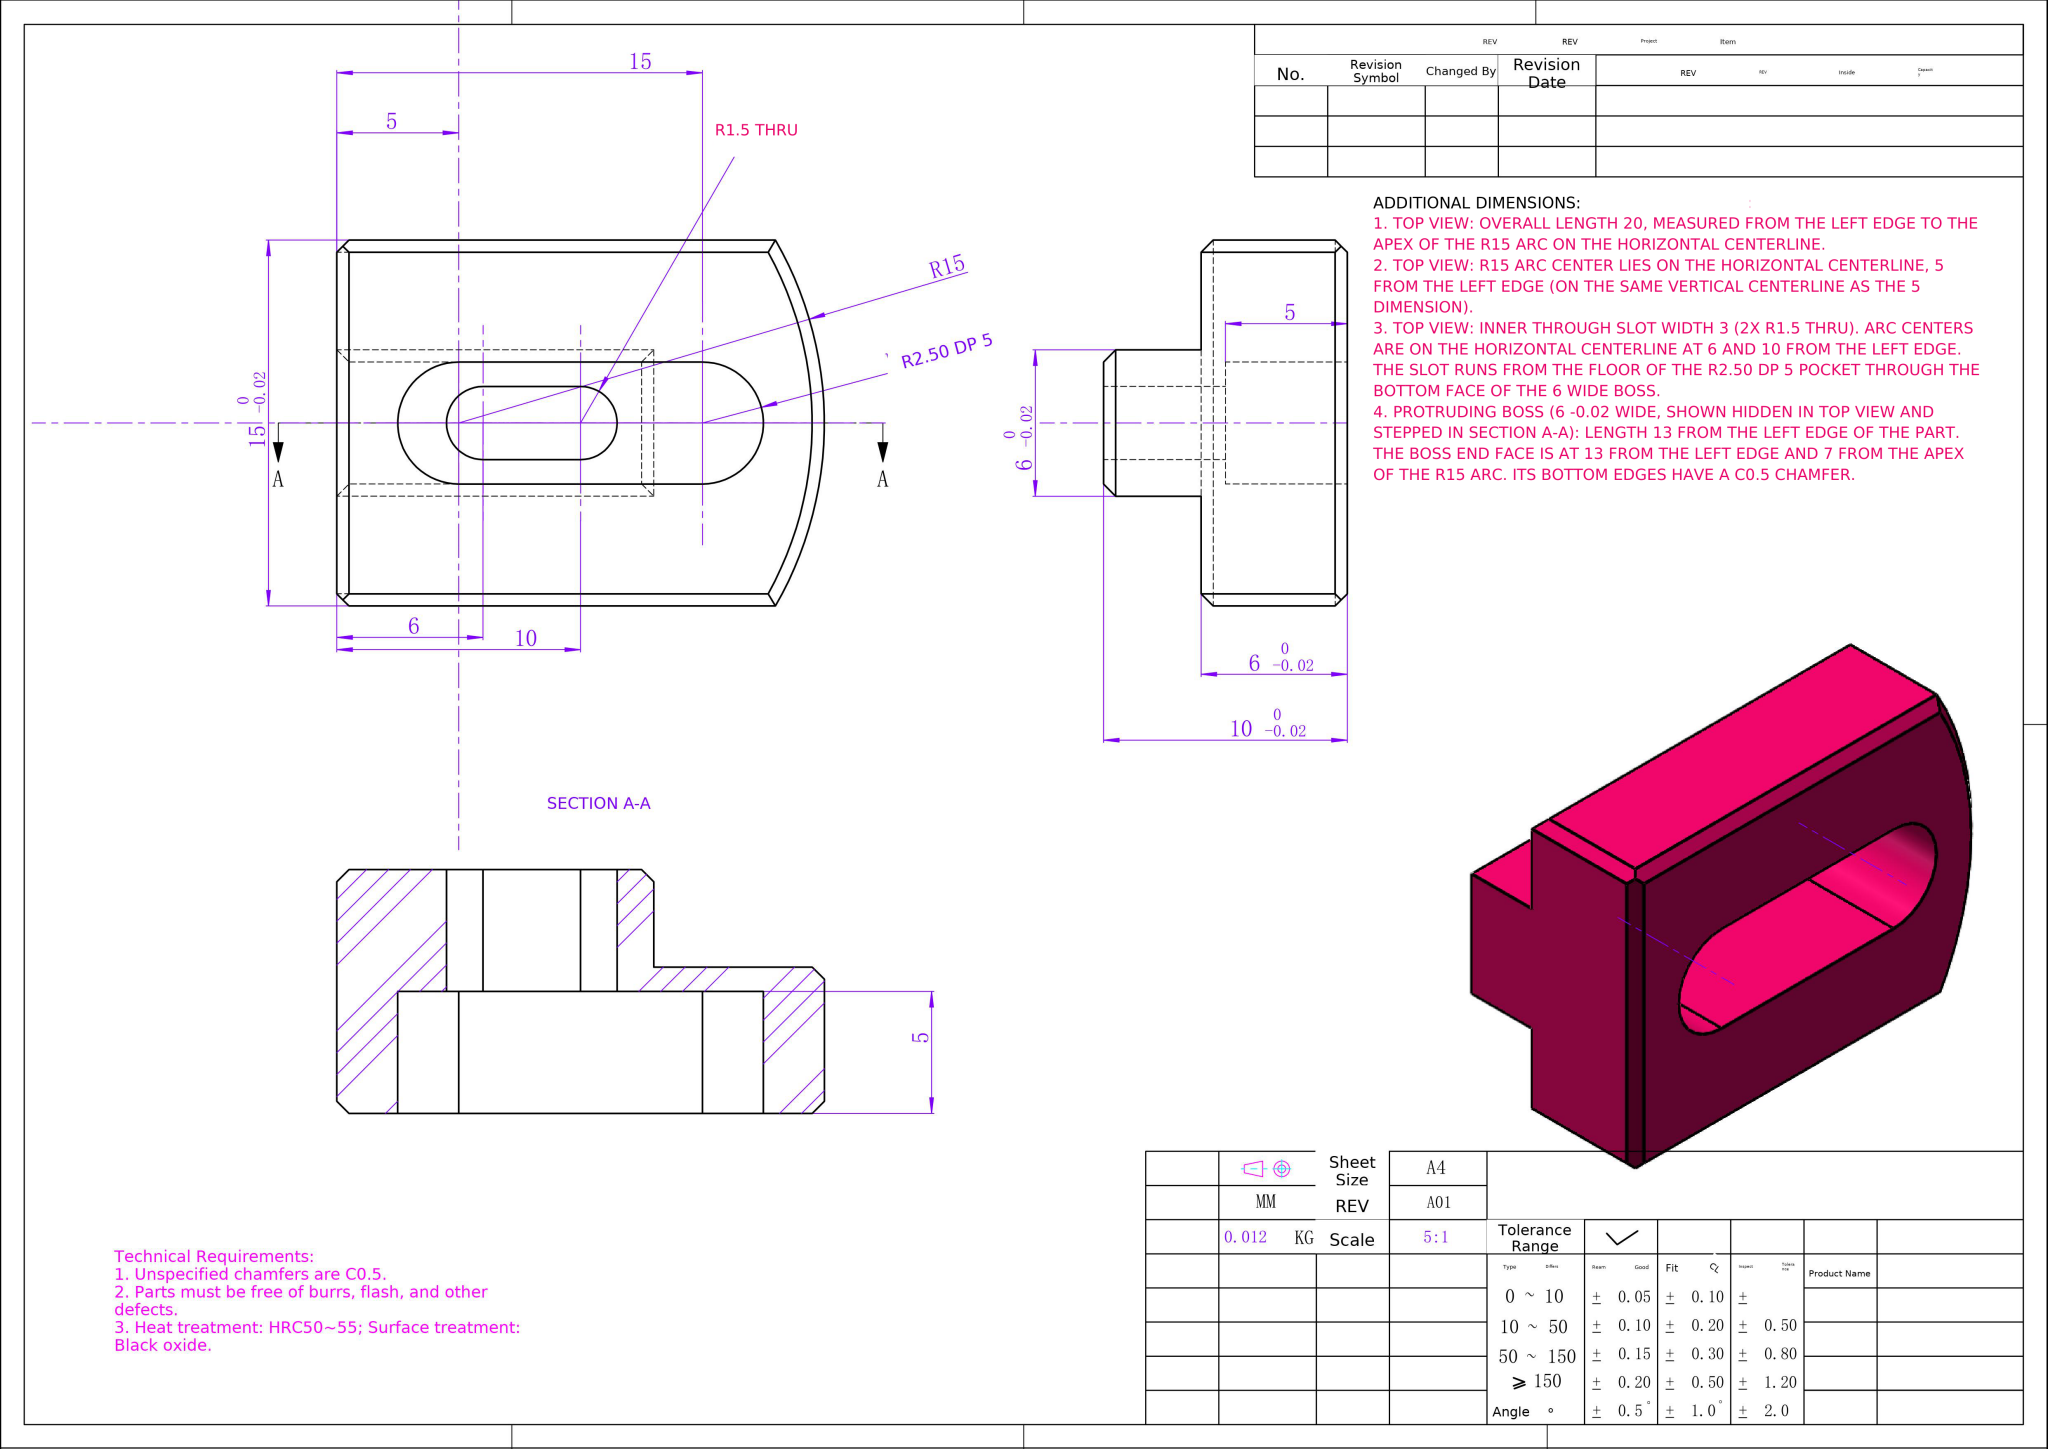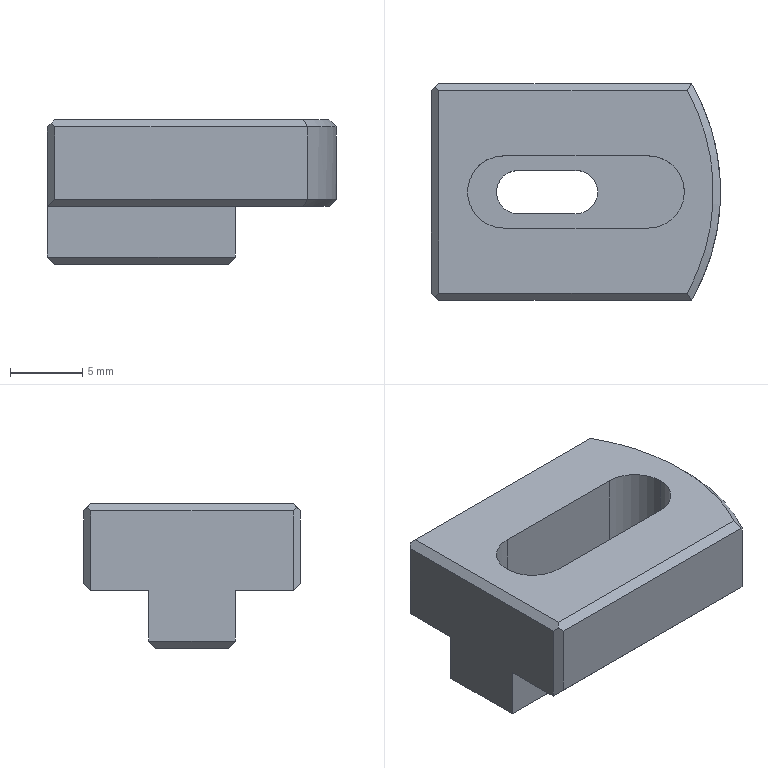Part | NX | mm | 1 solid | 35 faces | box 20 x 15 x 10 mm | volume 1589 mm3 | plane 25 | cylinder 7 | cone 3 | commonest cylinder face diameters 3 x3 5 x3 30 x1